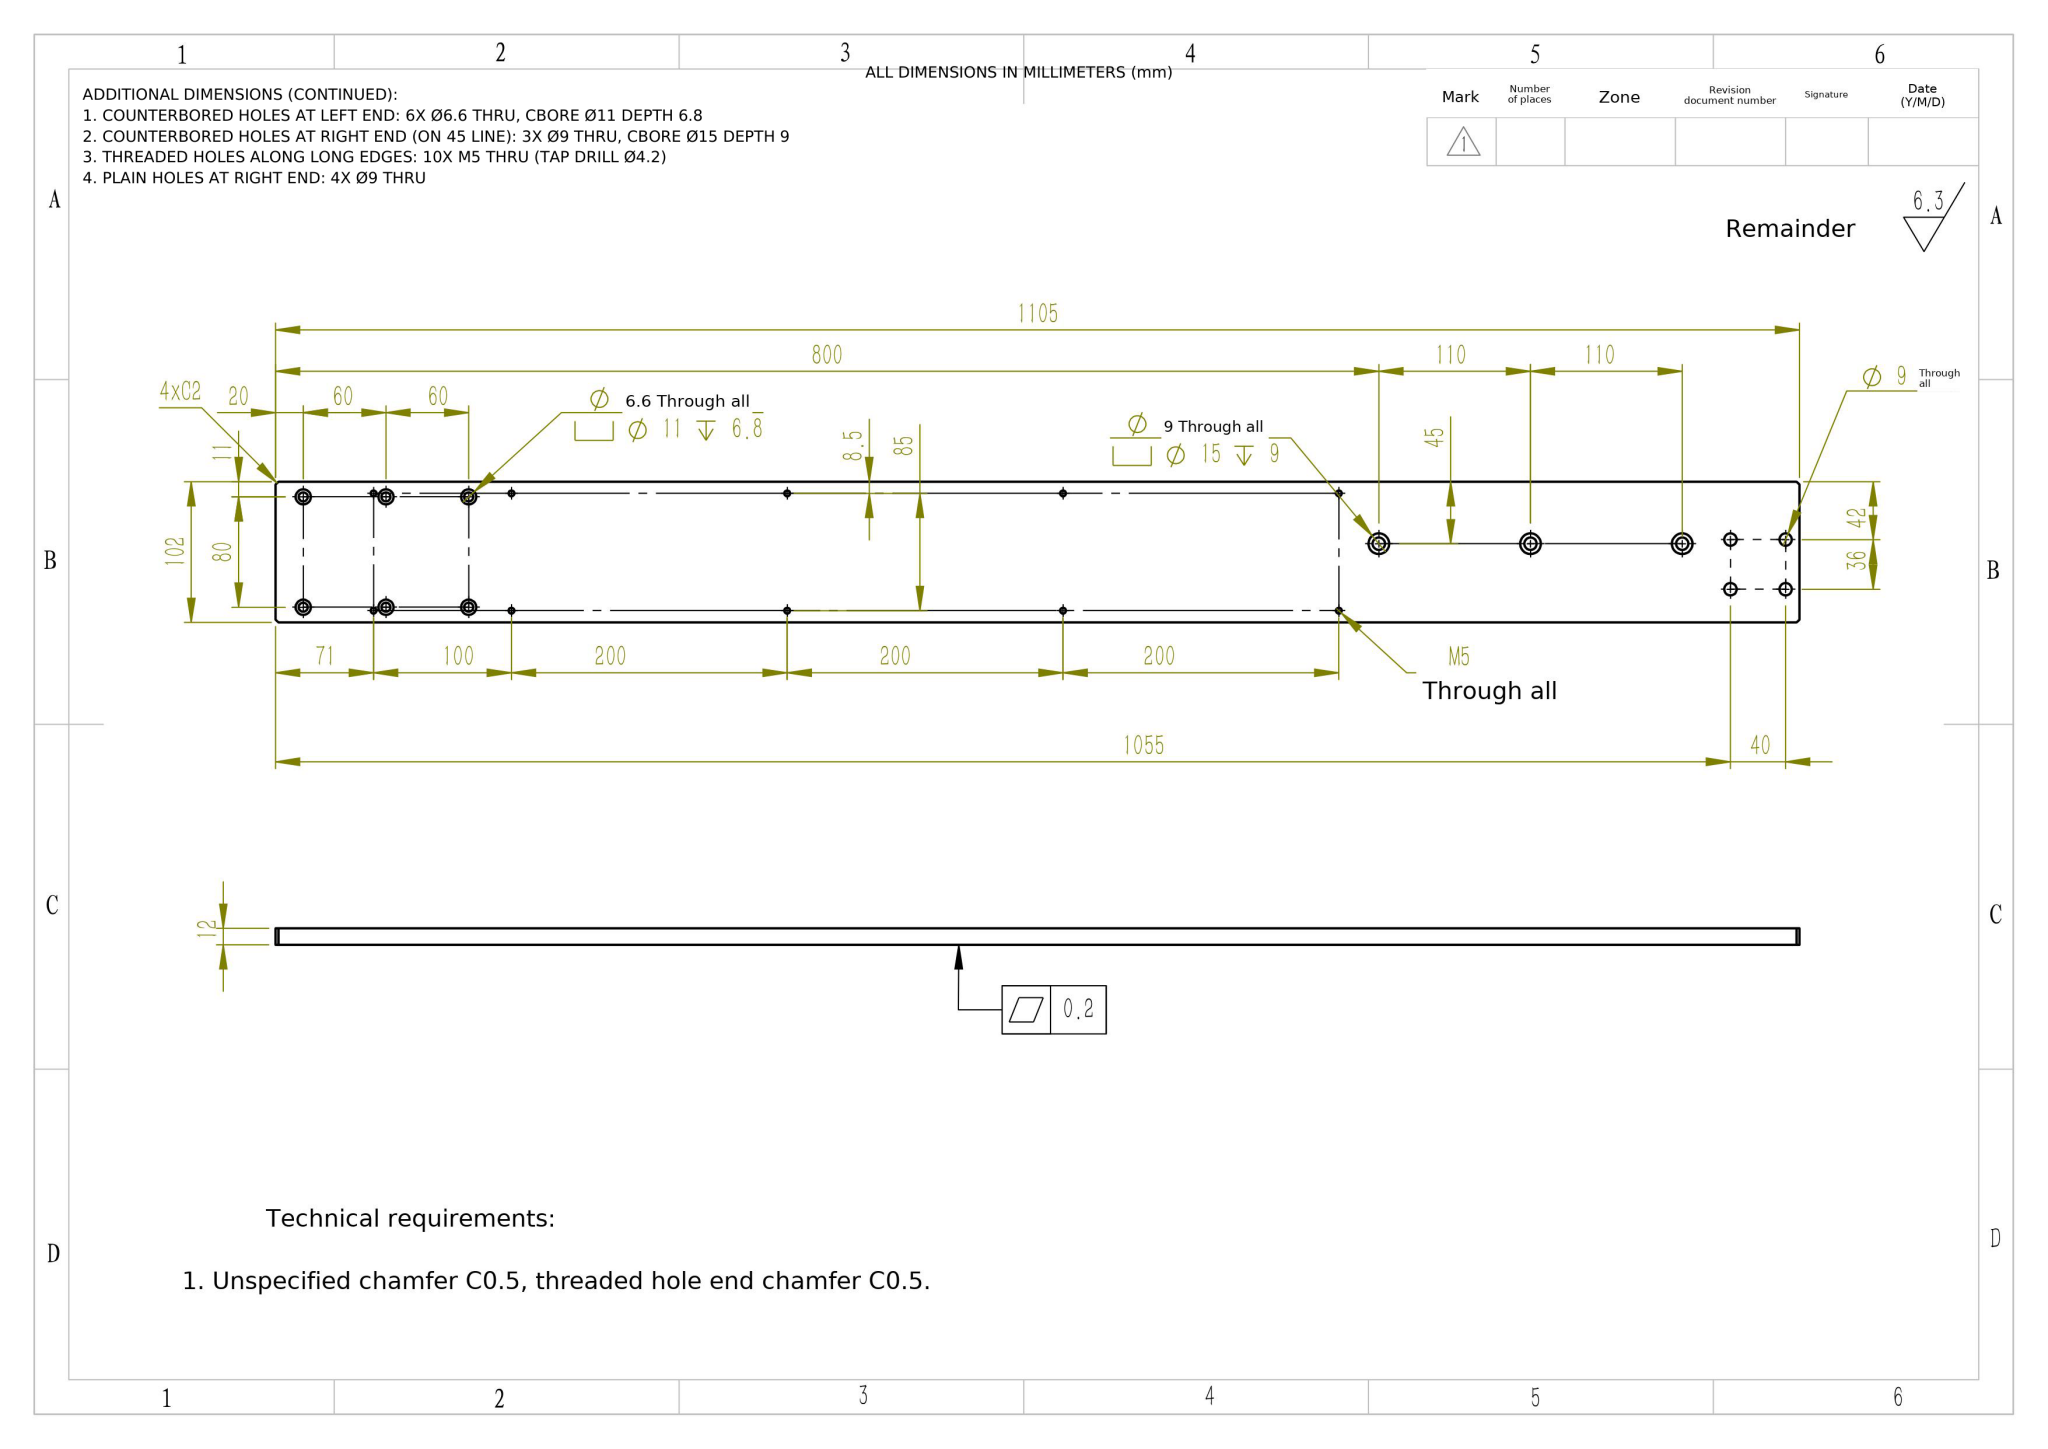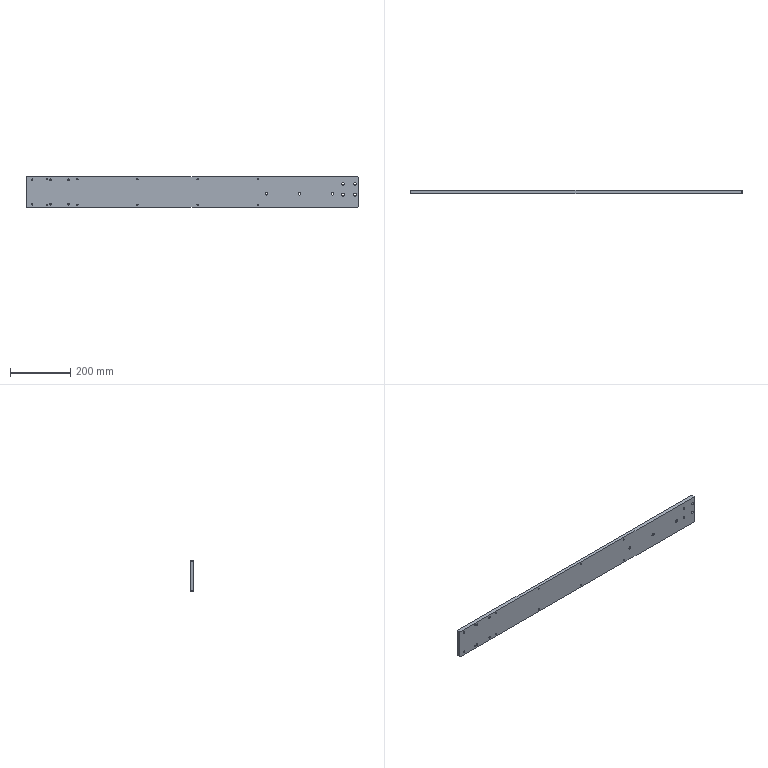Part | NX | mm | 1 solid | 83 faces | box 1105 x 12 x 102 mm | volume 1337419 mm3 | cylinder 64 | plane 19 | commonest cylinder face diameters 4.2 x20 9 x14 11 x12 6.6 x12 15 x6